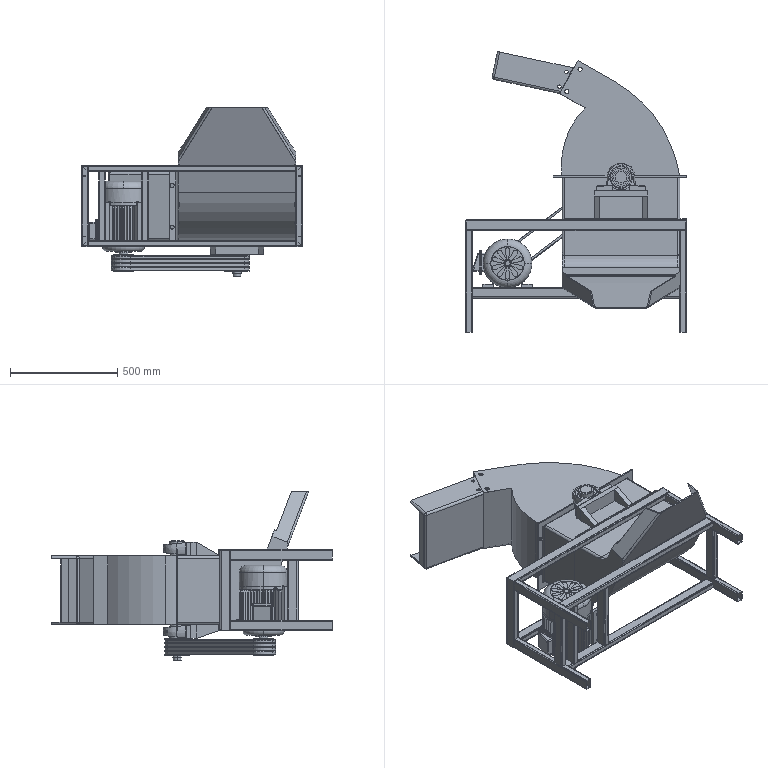Assembly | SolidWorks | mm | 76 component files | 78 solids | 1940 faces | box 1060 x 1310.75 x 790.04 mm | volume 31632157 mm3 | plane 992 | cylinder 640 | cone 226 | spline 70 | torus 12 | commonest cylinder face diameters 11.872 x72 10.4 x56 5.2 x56 227.5 x43 10 x22 10.5 x22 20 x19 21 x18
Bill of materials:
BearingHousing | 2 |  | Housing that looks like a pillow-block bearing: a rectangular base with two mounting lugs, a rounded body above it holding a ring insert with a cylindrical bore, and a small nipple-like protrusion on the rounded body.
Belt | 4 |  | Thin, flat closed loop shaped like a stadium (an elongated oval with straight sides and round ends) and a narrow rectangular cross-section.
DrivePulley | 1 |  | Cylindrical pulley-like wheel with several grooves: five rims separated by four V-shaped grooves around the outside, and a central bore with a keyway.
FeedInlet | 1 |  | Sheet-metal bracket bent into a C or U channel: a wide flat web with two parallel flanges at rounded bends, each flange having two small holes near its free edge.
SquareTube10 | 1 |  | Long straight hollow rectangular tube with rounded outer and inner corners and square-cut ends.
SquareTube1 | 1 |  | Long hollow rectangular tube with rounded corners and both ends cut at an angle (mitered), giving a trapezoid outline in one view.
SquareTube11 | 1 |  | Straight hollow rectangular tube with rounded corners and square-cut ends, shown standing vertically.
SquareTube12 | 1 |  | Straight hollow rectangular tube with rounded corners and square-cut ends, shown standing vertically.
SquareTube13 | 1 |  | Straight hollow rectangular tube with rounded corners and square-cut ends. It is vertical and looks slightly slimmer than parts 6 and 7.
SquareTube14 | 1 |  | Straight hollow rectangular tube with rounded corners and square-cut ends. It is vertical and looks slightly slimmer than parts 6 and 7.
SquareTube2 | 1 |  | Short hollow rectangular tube with rounded corners and both ends cut at parallel angles, giving a parallelogram outline in side view.
SquareTube3 | 1 |  | Long hollow rectangular tube with rounded corners and both ends mitered, so the outline is a trapezoid in one view. It looks similar to unnamed part, with the angled cuts facing the other way.
SquareTube4 | 1 |  | Straight length of thin-walled rectangular hollow tube with rounded corners. Both ends are cut at an angle (mitred).
SquareTube5 | 1 |  | Straight length of thin-walled rectangular hollow tube with rounded corners and square-cut ends.
SquareTube6 | 1 |  | Straight length of thin-walled rectangular hollow tube with rounded corners and square-cut ends.
SquareTube7 | 1 |  | Straight length of thin-walled rectangular hollow tube with rounded corners and square-cut ends.
SquareTube8 | 1 |  | Straight length of thin-walled rectangular hollow tube with rounded corners and square-cut ends.
SquareTube9 | 1 |  | Long, slender rectangular hollow tube with rounded corners and square-cut ends. Its section is wider and flatter than the other tubes, about 2:1.
Blade | 36 |  | Flat rectangular plate with sharp corners and one round through-hole near one end, centered across the width.
ToolHolder | 1 |  | Coaxial stack of six thin circular discs, evenly spaced, with a central cylinder (hub or spacer) between them. The discs have a central round bore with one rectangular keyway notch.
LowerHousing | 1 |  | Formed thin-sheet part. In side view it has a curved, J-like profile: a sloped straight leg that turns through a fillet into a flat section, with a large convex curve on the underside. It has angled side flanges, and a narrow bent lip at the end of the sloped leg.
MiddleHousing1 | 1 |  | Open rectangular sleeve or frame made of thin sheet: four walls enclosing a rectangular opening that runs through it. It has narrow edge flanges, a raised rectangular tab on the top wall, and a semicircular notch cut into the edge of one wall.
Stiffener | 1 |  | Solid wedge: a prism with a right-triangle profile and a small flat at the thin end, extruded to a uniform width.
Stiffener2 | 1 |  | Solid wedge: a prism with a right-triangle profile and a small flat at the thin end, extruded to a uniform width.
Stiffener3 | 1 |  | Solid wedge-shaped prismatic block: constant rectangular cross-section along its width, with a trapezoidal side profile where one long edge is inclined relative to the opposite edge.
Stiffener4 | 1 |  | Solid wedge-shaped prismatic block with a trapezoidal side profile and rectangular end/top projections; same geometry as unnamed part.
ParallelKey | 1 |  | Flat elongated bar with fully rounded (semicircular) ends and slightly rounded edges, giving an obround outline; shape resembles a round-ended key.
ParallelKey20_220_12 | 1 |  | Thin, long flat bar with rounded ends (obround outline) and small edge rounds; narrower and thinner than the similar bars in this set.
ParallelKey4_70 | 1 |  | Flat elongated bar with semicircular ends and lightly rounded edges (obround outline); proportions sit between the other two rounded-end bars.
Pulley | 1 |  | Multi-groove sheave/pulley: cylindrical body with five rims separating four V-shaped circumferential grooves, a central bore with a single keyway, four axial through holes around the bore, and a recessed face with a raised hub ring.
Spindle | 1 |  | Stepped cylindrical shaft with several coaxial diameter sections: a short end journal, a long larger-diameter main section, and progressively smaller sections toward the other end, with small chamfers/rounds at the steps.
Motor | 1 |  | Cylindrical finned housing body: a central cylinder with many longitudinal radial fins, a domed cylindrical cover on one end, a smaller protruding shaft on the opposite end, and a rectangular box projecting from one side; the overall form resembles an electric motor.
MotorJunctionBox | 1 |  | Box-like body on a rectangular rounded-corner flange; the body has a tapered (trapezoidal) side profile, filleted edges, and four through holes near the flange corners.
MotorMount | 1 |  | Rectangular flat bar/plate with two circular through holes located near each end along the centerline.
MotorMountBasePlate | 1 |  | Rectangular flat bar/plate with two circular through holes near each end; the holes appear slightly offset from the width centerline.
MotorProtectiveCover | 1 |  | Thin-walled cylindrical cap with a domed/rounded closed end containing a central round hole surrounded by about ten radial teardrop-shaped slots; the open rim has small notches and small round holes.
UpperHousing1 | 1 |  | Thin-walled, sheet-like curved housing or duct-bend shape. It has two parallel fan-shaped (circular-sector) plates joined by a curved outer wall. One straight side is open and surrounded by a flat rectangular frame flange with holes. An angled tab with two holes sticks out from the plate edge on the far side.
Mates: